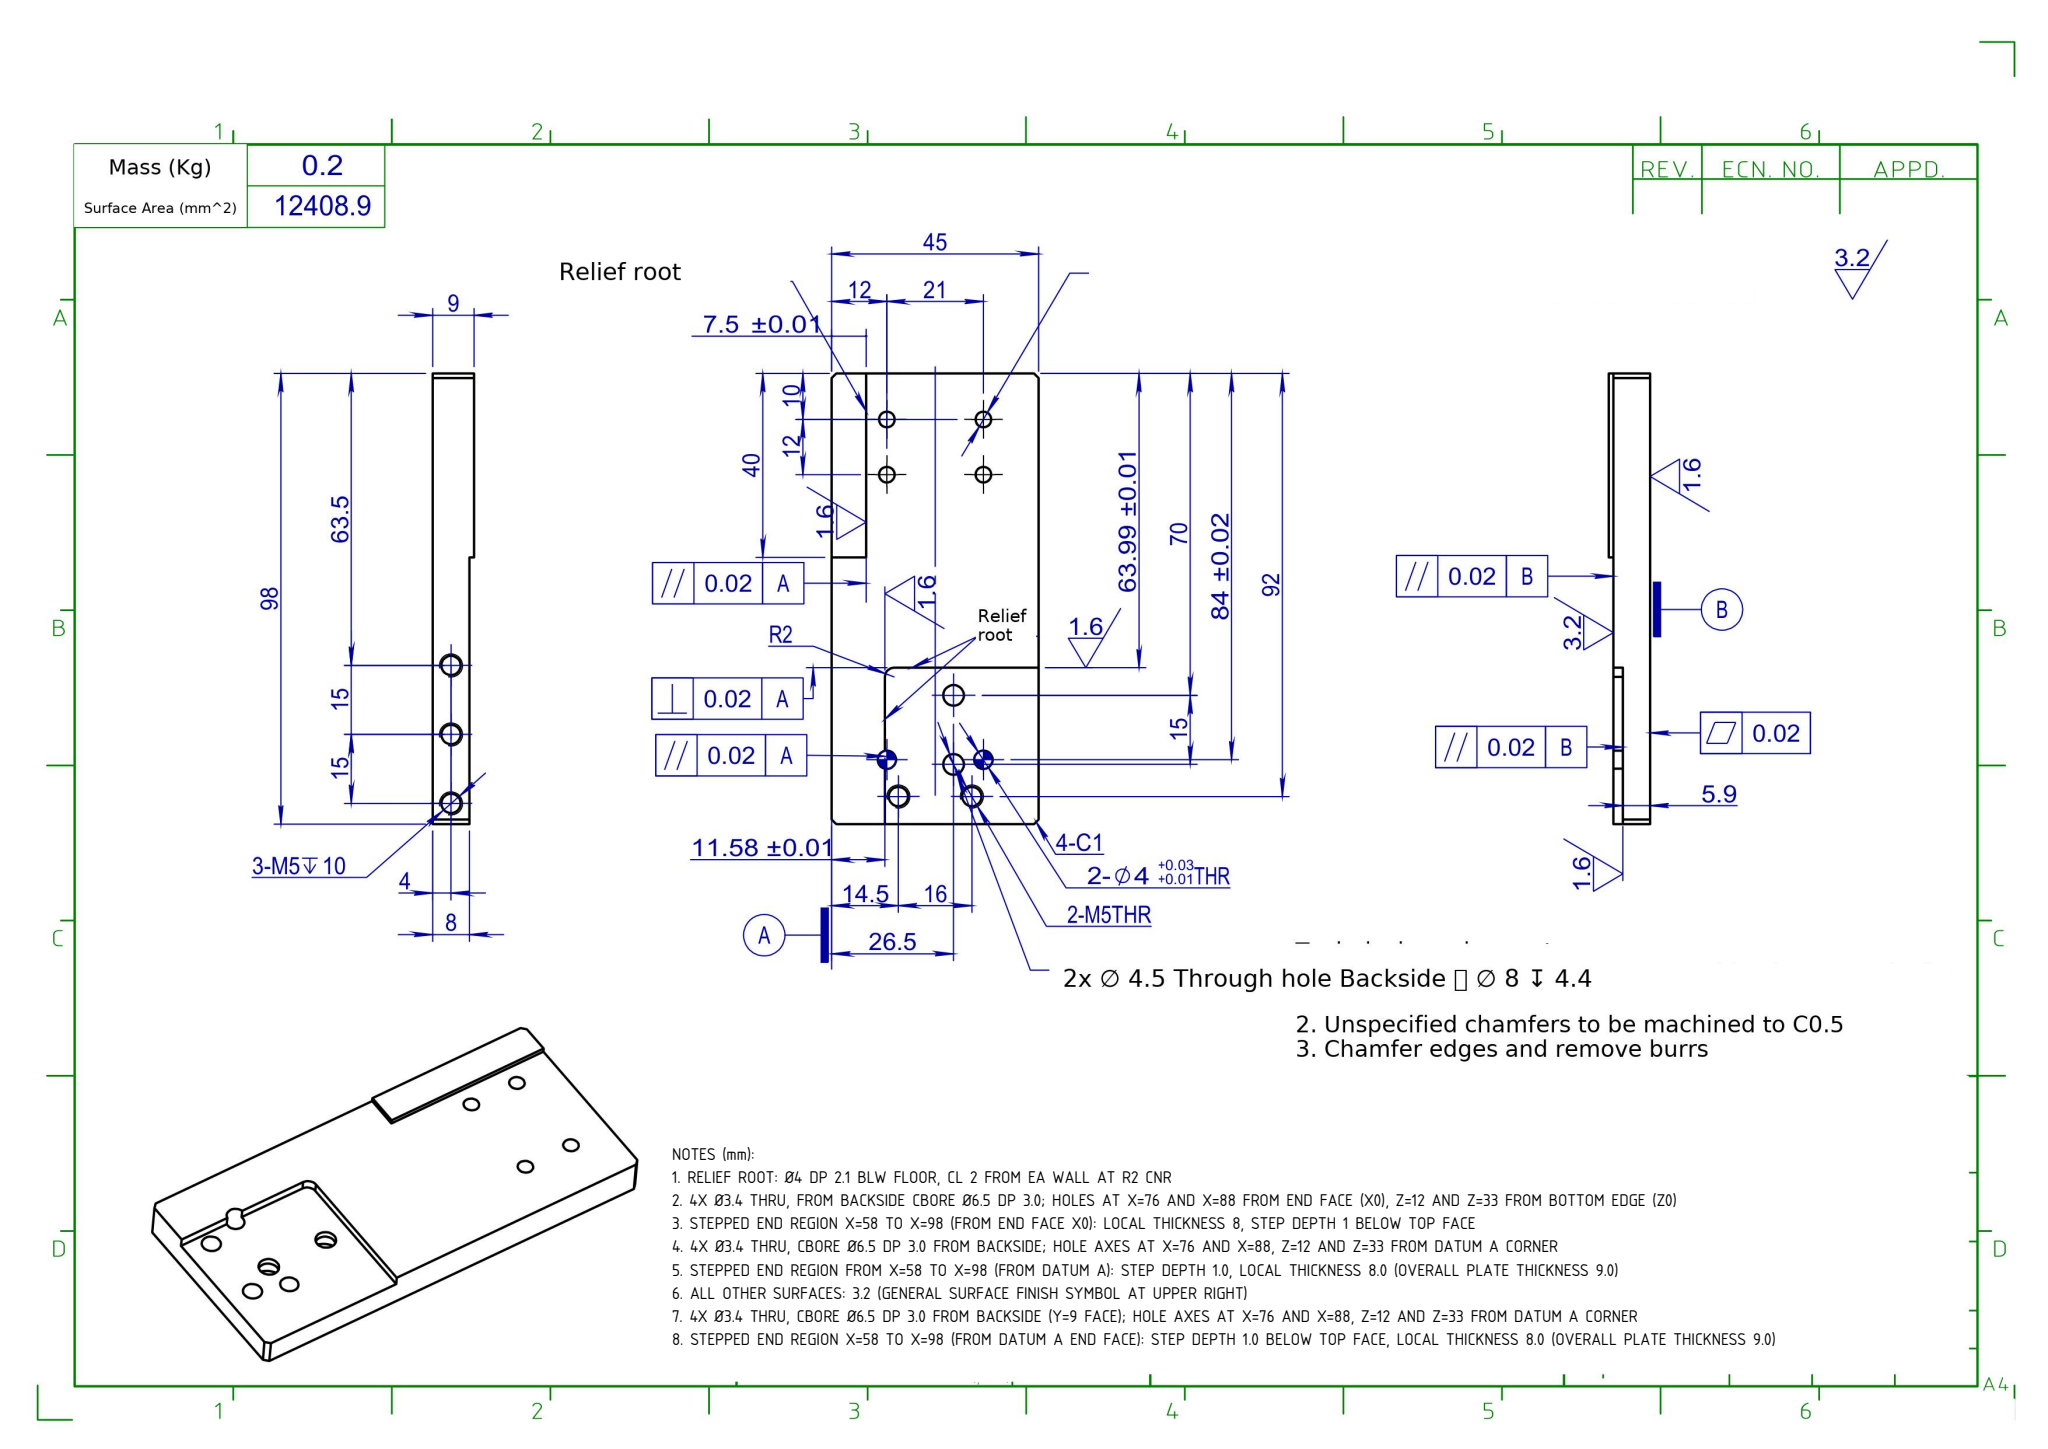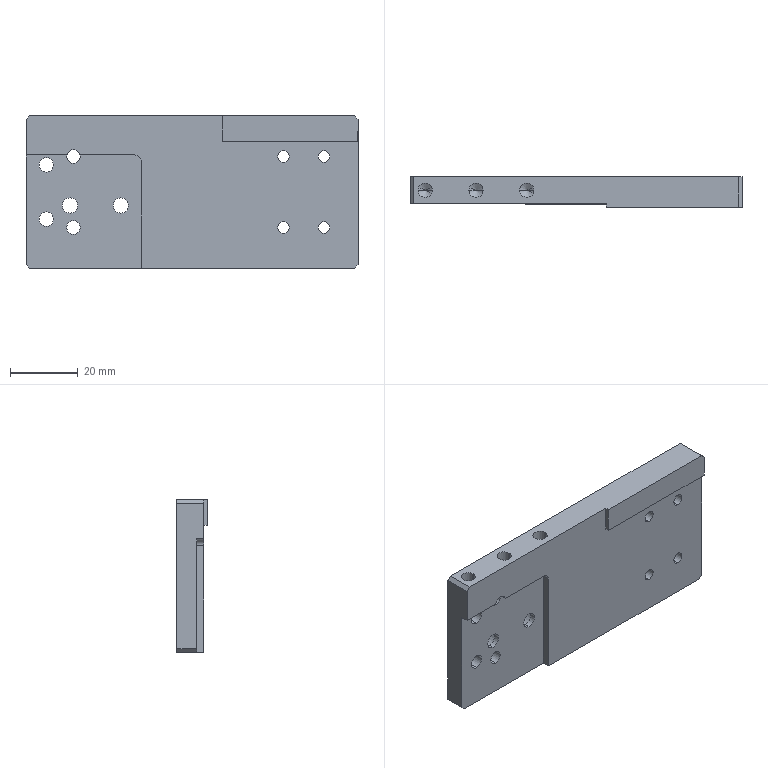Part | SolidWorks | mm | 1 solid | 68 faces | box 98 x 9 x 45 mm | volume 31314 mm3 | cylinder 39 | plane 23 | cone 6 | commonest cylinder face diameters 4.2 x10 6.5 x8 3.4 x8 4 x5 8 x4 4.5 x4
Drawing notes:
RELIEF ROOT: Ø4 DP 2.1 BLW FLOOR, CL 2 FROM EA WALL AT R2 CNR | from the solid: Cyl Ø4 axis y at (x=32.01, z=31.42) len 2.1; pocket walls x=34.01 & z=33.42 give CL offset 2 from each; y planes 3.1 to 1.0 = 2.1 deep
4X Ø3.4 THRU, FROM BACKSIDE CBORE Ø6.5 DP 3.0; HOLES AT X=76 AND X=88 FROM END FACE (X0), Z=12 AND Z=33 FROM BOTTOM EDGE (Z0) | from the solid: cylinders dia 3.4 axis y at (76,12),(76,33),(88,12),(88,33) len 5.0 and matching dia 6.5 axis y same positions len 3.0
STEPPED END REGION X=58 TO X=98 (FROM END FACE X0): LOCAL THICKNESS 8, STEP DEPTH 1 BELOW TOP FACE | from the solid: axis_planes x=58.0 and x=98.0; y plane at 1.0 with bbox y height 9.0 (9-1=8 local thickness, 1 step depth)
4X Ø3.4 THRU, CBORE Ø6.5 DP 3.0 FROM BACKSIDE; HOLE AXES AT X=76 AND X=88, Z=12 AND Z=33 FROM DATUM A CORNER | from the solid: cylinders 3.4 dia, axis y, at (76,12),(76,33),(88,12),(88,33) len 5.0 and cylinders 6.5 dia, axis y, same 4 positions, len 3.0
STEPPED END REGION FROM X=58 TO X=98 (FROM DATUM A): STEP DEPTH 1.0, LOCAL THICKNESS 8.0 (OVERALL PLATE THICKNESS 9.0) | from the solid: axis_planes x=58.0 and y=1.0 with bbox_xyz y=9.0
ALL OTHER SURFACES: 3.2 (GENERAL SURFACE FINISH SYMBOL AT UPPER RIGHT) | from the solid: no STEP geometry; restores text lost by redaction of the overlapped callout
4X Ø3.4 THRU, CBORE Ø6.5 DP 3.0 FROM BACKSIDE (Y=9 FACE); HOLE AXES AT X=76 AND X=88, Z=12 AND Z=33 FROM DATUM A CORNER | from the solid: cylinders: Ø3.4 y-axis holes at (x76,z12),(x76,z33),(x88,z12),(x88,z33) from y=1.0 to 6.0; coaxial Ø6.5 bores same 4 axes from y=6.0 to 9.0; planes y=6.0 cbore floors (4x)
STEPPED END REGION X=58 TO X=98 (FROM DATUM A END FACE): STEP DEPTH 1.0 BELOW TOP FACE, LOCAL THICKNESS 8.0 (OVERALL PLATE THICKNESS 9.0) | from the solid: axis_planes: y=0.0 face extent x[58,98] z[37.5,45]; y=1.0 face extent x[0,98] z[0,45]; bbox_xyz y=9.0; plane x=58 extent y[0,1]
build123d program:
from build123d import *

# Parameters (mm, degrees)
SKETCH1_W                                            = 98
SKETCH1_H                                            = 45
EXTRUDE1_DEPTH                                       = 8
COUNTERBORE_FOR_M3_HEX_SOCKET_HEAD_CAP_S_D           = 3.4
COUNTERBORE_FOR_M3_HEX_SOCKET_HEAD_CAP_S_CBORE_D     = 6.5
COUNTERBORE_FOR_M3_HEX_SOCKET_HEAD_CAP_S_CBORE_DEPTH = 3
SKETCH9_W                                            = 40
SKETCH9_H                                            = 7.5
EXTRUDE2_DEPTH                                       = 1
SKETCH17_W                                           = 50
SKETCH17_H                                           = 45
CUT_EXTRUDE5_DEPTH                                   = 2.1
COUNTERBORE_FOR_M4_HEX_SOCKET_HEAD_CAP_S_D           = 4.5
COUNTERBORE_FOR_M4_HEX_SOCKET_HEAD_CAP_S_CBORE_D     = 8
COUNTERBORE_FOR_M4_HEX_SOCKET_HEAD_CAP_S_CBORE_DEPTH = 4.4
SKETCH20_W                                           = 34.006
SKETCH20_H                                           = 11.576
BOSS_EXTRUDE1_DEPTH                                  = 2.1
FILLET1_R                                            = 2
M5_TAPPED_HOLE2_D                                    = 4.2
SKETCH28_R                                           = 2
CUT_EXTRUDE9_DEPTH                                   = 55.665
CHAMFER3_SIZE                                        = 1
M5_TAPPED_HOLE1_D                                    = 4.2
M5_TAPPED_HOLE1_DEPTH                                = 11
M5_TAPPED_HOLE1_TIP                                  = 1.262


with BuildPart() as part:
    # Sketch1 → Extrude1 (new body)
    with BuildSketch(Plane(origin=(0, 0, 0), x_dir=(1, 0, 0), z_dir=(0, 1, 0))):
        Rectangle(SKETCH1_W, SKETCH1_H)
    extrude(amount=EXTRUDE1_DEPTH)

    # Counterbore for M3 Hex Socket Head Cap S (through all)
    with Locations(Plane(origin=(0, 8, 0), x_dir=(-1, 0, 0), z_dir=(0, 1, 0))):
        with Locations((-39, -10.5), (-39, 10.5), (-27, -10.5), (-27, 10.5)):
            CounterBoreHole(COUNTERBORE_FOR_M3_HEX_SOCKET_HEAD_CAP_S_D / 2, COUNTERBORE_FOR_M3_HEX_SOCKET_HEAD_CAP_S_CBORE_D / 2, COUNTERBORE_FOR_M3_HEX_SOCKET_HEAD_CAP_S_CBORE_DEPTH)

    # Sketch9 → Extrude2 (add)
    with BuildSketch(Plane.XZ):
        with Locations((29, 18.75)):
            Rectangle(SKETCH9_W, SKETCH9_H)
    extrude(amount=EXTRUDE2_DEPTH)

    # Sketch17 → Cut-Extrude5 (cut)
    with BuildSketch(Plane(origin=(0, 0, 0), x_dir=(-1, 0, 0), z_dir=(0, -1, 0))):
        with Locations((39.994, 0)):
            Rectangle(SKETCH17_W, SKETCH17_H)
    extrude(amount=-CUT_EXTRUDE5_DEPTH, mode=Mode.SUBTRACT)

    # Counterbore for M4 Hex Socket Head Cap S (through all)
    with Locations(Plane(origin=(0, 8, 0), x_dir=(1, 0, 0), z_dir=(0, 1, 0))):
        with Locations((-21, 4), (-36, 4)):
            CounterBoreHole(COUNTERBORE_FOR_M4_HEX_SOCKET_HEAD_CAP_S_D / 2, COUNTERBORE_FOR_M4_HEX_SOCKET_HEAD_CAP_S_CBORE_D / 2, COUNTERBORE_FOR_M4_HEX_SOCKET_HEAD_CAP_S_CBORE_DEPTH)

    # Sketch20 → Boss-Extrude1 (add)
    with BuildSketch(Plane.XZ.offset(-2.1)):
        with Locations((-31.997, 16.712)):
            Rectangle(SKETCH20_W, SKETCH20_H)
    extrude(amount=BOSS_EXTRUDE1_DEPTH)

    # Fillet1
    fillet1_edges = [part.edges().sort_by_distance(p)[0] for p in [
        (-14.994, 1.05, 10.924),
    ]]
    fillet(fillet1_edges, radius=FILLET1_R)

    # M5 Tapped Hole2 (through all)
    with Locations(Plane(origin=(0, 8, 0), x_dir=(1, 0, 0), z_dir=(0, 1, 0))):
        with Locations((-43, -8), (-43, 8)):
            Hole(M5_TAPPED_HOLE2_D / 2)

    # Sketch28 → Cut-Extrude9 (cut, through all)
    with BuildSketch(Plane(origin=(0, 8, 0), x_dir=(1, 0, 0), z_dir=(0, 1, 0))):
        with Locations(Location((-35, -10.5, 0), (0, 0, 270))):
            Circle(SKETCH28_R)
        with Locations(Location((-35, 10.5, 0), (0, 0, 270))):
            Circle(SKETCH28_R)
    extrude(amount=-CUT_EXTRUDE9_DEPTH, mode=Mode.SUBTRACT)

    # Chamfer3
    chamfer3_edges = [part.edges().sort_by_distance(p)[0] for p in [
        (-49, 4, 22.5),
        (-49, 5.05, -22.5),
        (49, 4, -22.5),
        (49, 3.5, 22.5),
    ]]
    chamfer(chamfer3_edges, length=CHAMFER3_SIZE)

    # M5 Tapped Hole1
    with Locations(Plane.XY.offset(22.5)):
        with Locations((-44.5, 4), (-29.5, 4), (-14.5, 4)):
            Hole(M5_TAPPED_HOLE1_D / 2, depth=M5_TAPPED_HOLE1_DEPTH)
            with Locations((0, 0, -(M5_TAPPED_HOLE1_DEPTH + M5_TAPPED_HOLE1_TIP / 2))):  # 118° drill point
                Cone(0, M5_TAPPED_HOLE1_D / 2, M5_TAPPED_HOLE1_TIP, mode=Mode.SUBTRACT)


solid = part.part